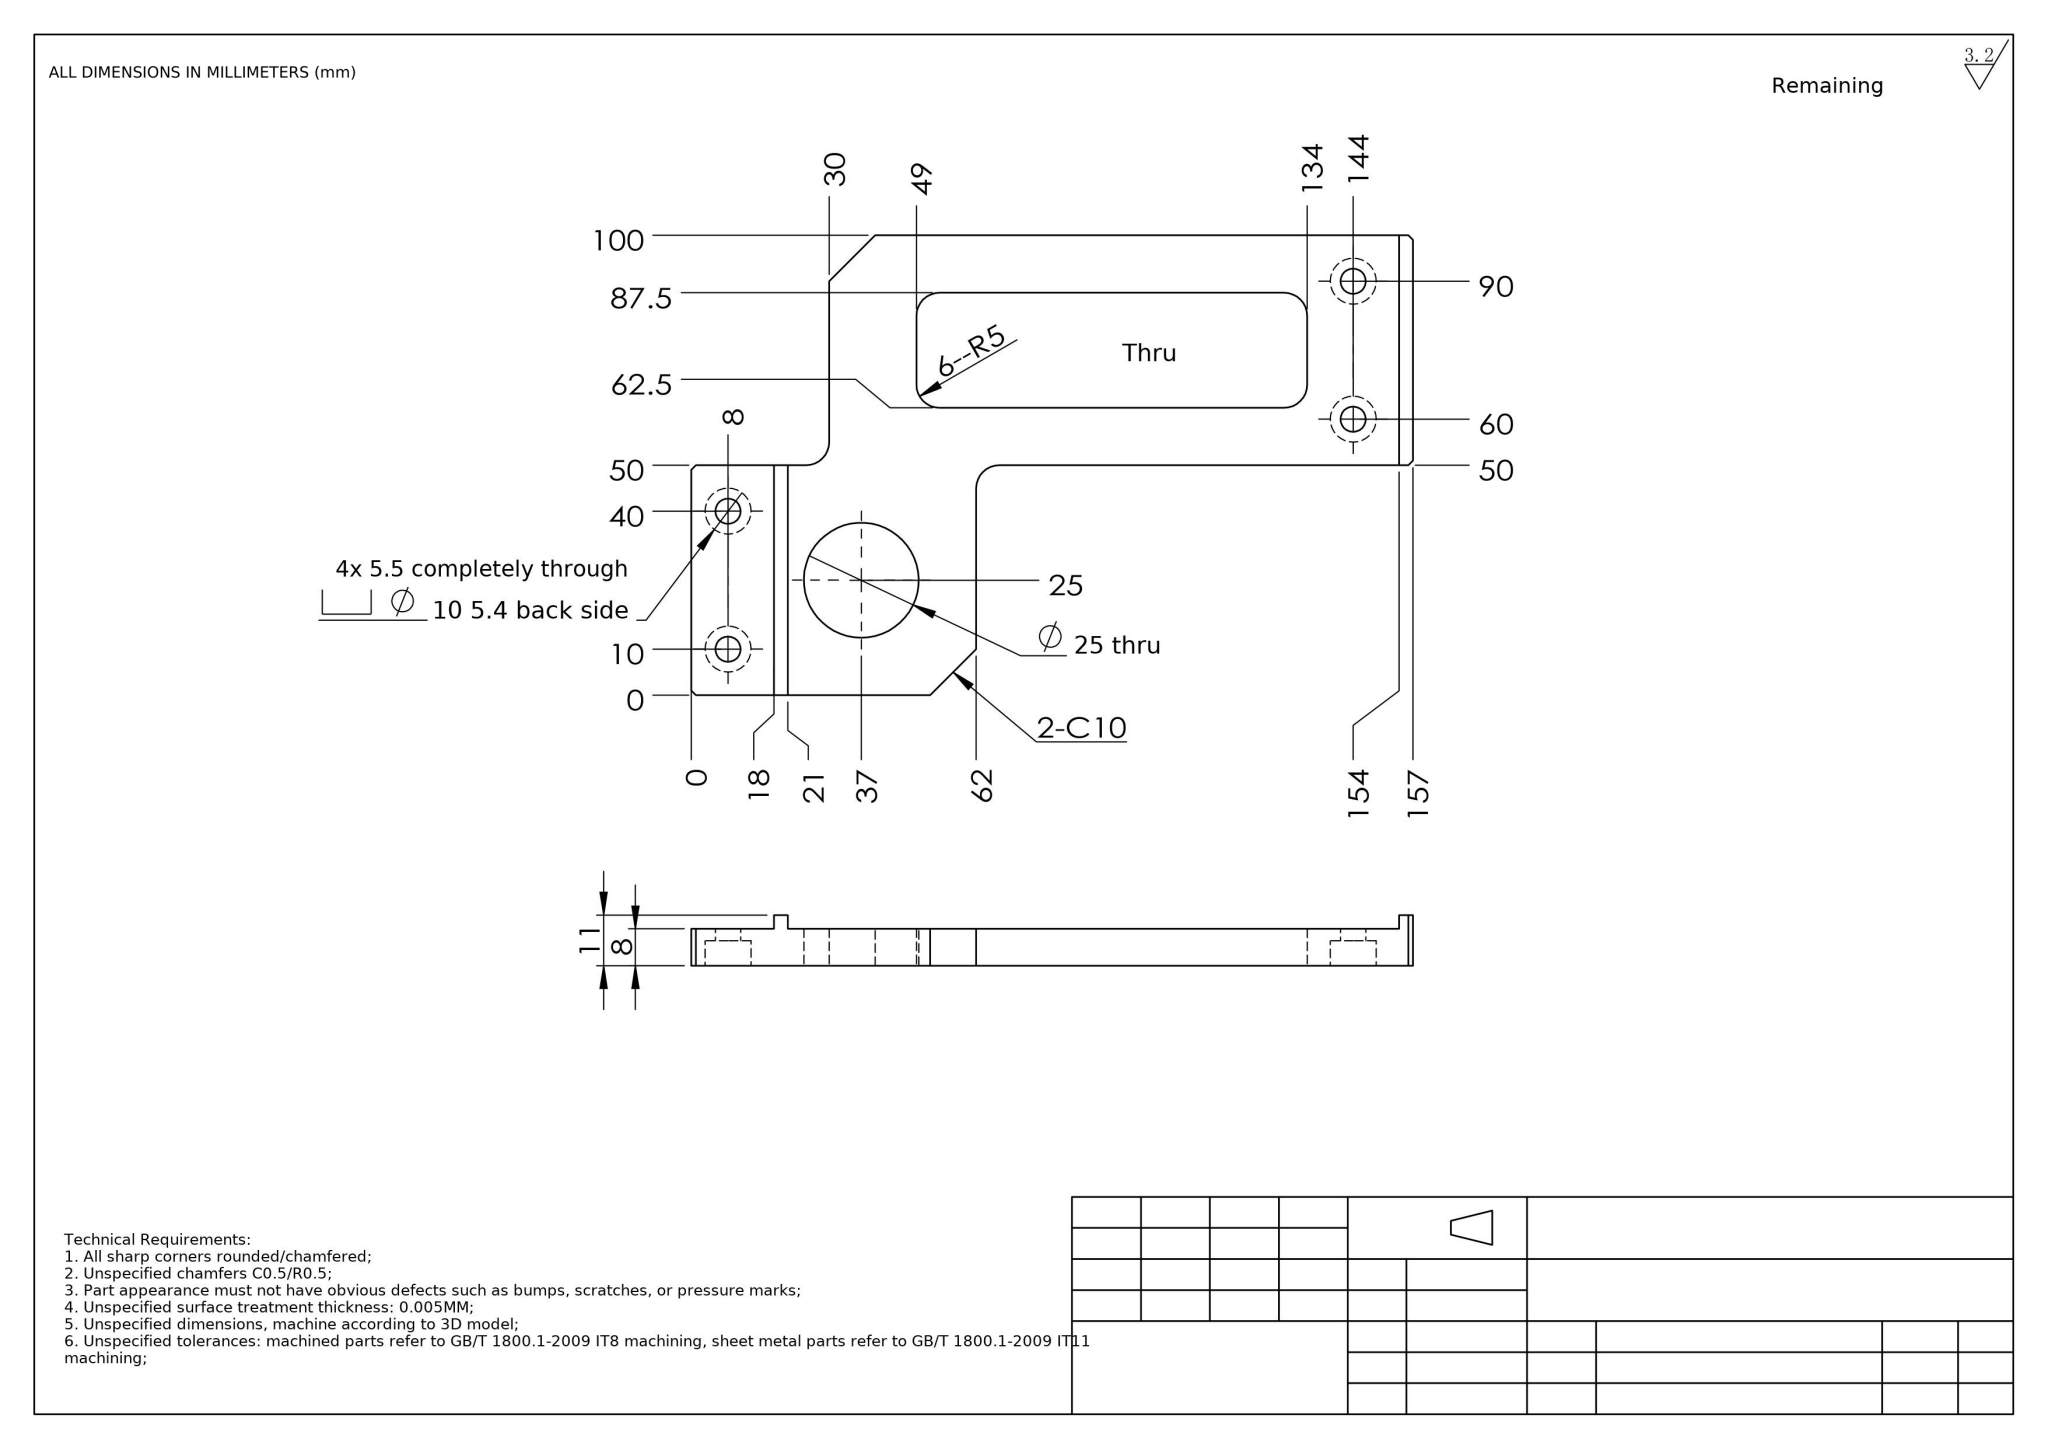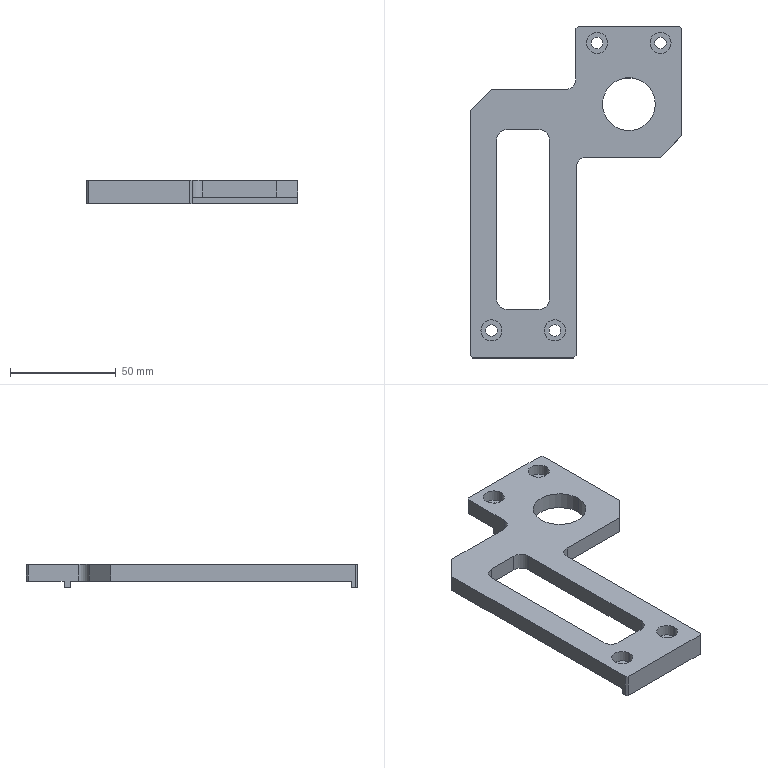Part | NX | mm | 1 solid | 54 faces | box 100 x 157 x 11 mm | volume 53068 mm3 | plane 30 | cylinder 24 | commonest cylinder face diameters 10 x14 5.5 x8 25 x2